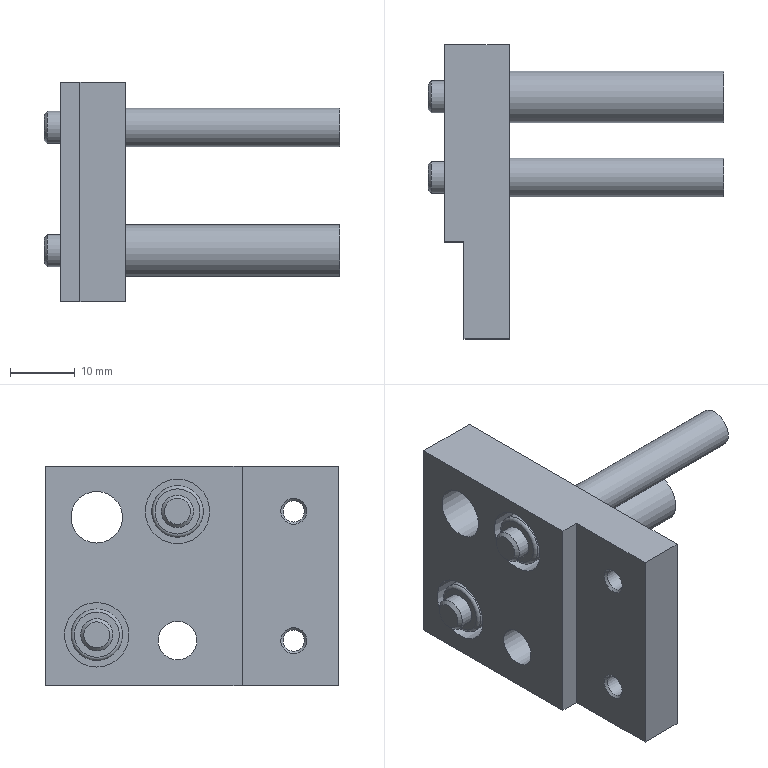Component | NX | AUX_CLAMP_CYL_COMP | 1 solid | 36 faces | volume 15397 mm3 | plane 16 | cylinder 12 | cone 6 | torus 2 | commonest cylinder face diameters 8 x4 10 x2 6 x2 5 x2 3.3 x2